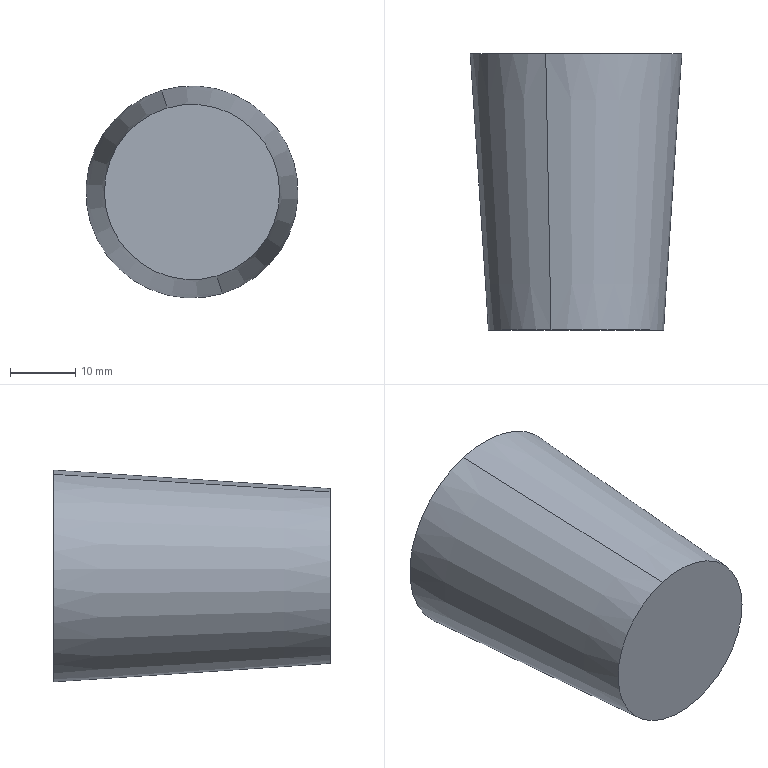Component | SolidWorks | CoffeeCup-1 | 1 solid | 7 faces | box 32.54 x 42.38 x 32.54 mm | volume 8227 mm3 | cone 4 | plane 3
build123d program:
from build123d import *

# Parameters (mm, degrees)
SHELL1_T = -2


with BuildPart() as part:
    # Sketch1 → Revolve1 (revolve)
    with BuildSketch(Plane.XY, mode=Mode.PRIVATE) as revolve1_sk:
        Polygon((0, 0), (16.271, 0), (13.443, -42.384), (0, -42.384), align=None)
    revolve(revolve1_sk.sketch.rotate(Axis((0, -42.384, 0), (0, 1, 0)), 90), axis=Axis((0, -42.384, 0), (0, 1, 0)))

    # Shell1
    shell1_openings = [part.faces().sort_by_distance(p)[0] for p in [
        (0, 0, 0),
    ]]
    offset(amount=SHELL1_T, openings=shell1_openings, kind=Kind.INTERSECTION)


solid = part.part

# Placed as in the assembly
solid = solid.moved(Location((-79.558, -23.012, 243.54), (0, 0, 0)))
STEP:
#1=CARTESIAN_POINT('',(-3.262,-2.496,10.025));
#2=VERTEX_POINT('',#1);
#3=CARTESIAN_POINT('',(-3.002,-2.496,9.152));
#4=VERTEX_POINT('',#3);
#5=CARTESIAN_POINT('',(-3.132,-2.496,9.588));
#6=DIRECTION('',(0.,-1.,0.));
#7=DIRECTION('',(0.2855,0.,-0.9584));
#8=AXIS2_PLACEMENT_3D('',#5,#6,#7);
#9=CIRCLE('',#8,0.4556);
#10=EDGE_CURVE('',#2,#4,#9,.T.);
#11=ORIENTED_EDGE('',*,*,#10,.T.);
#12=CARTESIAN_POINT('',(-2.972,-0.906,9.05));
#13=VERTEX_POINT('',#12);
#14=CARTESIAN_POINT('',(-3.004,-2.569,9.156));
#15=DIRECTION('',(0.01901,0.9978,-0.06379));
#16=VECTOR('',#15,39.37);
#17=LINE('',#14,#16);
#18=EDGE_CURVE('',#4,#13,#17,.T.);
#19=ORIENTED_EDGE('',*,*,#18,.T.);
#20=CARTESIAN_POINT('',(-3.293,-0.906,10.126));
#21=VERTEX_POINT('',#20);
#22=CARTESIAN_POINT('',(-3.132,-0.906,9.588));
#23=DIRECTION('',(0.,-1.,0.));
#24=DIRECTION('',(-0.2855,0.,0.9584));
#25=AXIS2_PLACEMENT_3D('',#22,#23,#24);
#26=CIRCLE('',#25,0.5617);
#27=EDGE_CURVE('',#21,#13,#26,.T.);
#28=ORIENTED_EDGE('',*,*,#27,.F.);
#29=CARTESIAN_POINT('',(-3.261,-2.569,10.02));
#30=DIRECTION('',(-0.01901,0.9978,0.06379));
#31=VECTOR('',#30,39.37);
#32=LINE('',#29,#31);
#33=EDGE_CURVE('',#2,#21,#32,.T.);
#34=ORIENTED_EDGE('',*,*,#33,.F.);
#35=EDGE_LOOP('',(#11,#19,#28,#34));
#36=FACE_OUTER_BOUND('',#35,.T.);
#37=CARTESIAN_POINT('',(-3.132,-2.569,9.588));
#38=DIRECTION('',(0.,1.,0.));
#39=DIRECTION('',(-0.2855,0.,0.9584));
#40=AXIS2_PLACEMENT_3D('',#37,#38,#39);
#41=CONICAL_SURFACE('',#40,0.4507,0.06661);
#42=ADVANCED_FACE('',(#36),#41,.F.);
#43=CARTESIAN_POINT('',(-2.981,-2.575,9.081));
#44=VERTEX_POINT('',#43);
#45=CARTESIAN_POINT('',(-3.283,-2.575,10.095));
#46=VERTEX_POINT('',#45);
#47=CARTESIAN_POINT('',(-3.132,-2.575,9.588));
#48=DIRECTION('',(0.,-1.,0.));
#49=DIRECTION('',(0.2855,0.,-0.9584));
#50=AXIS2_PLACEMENT_3D('',#47,#48,#49);
#51=CIRCLE('',#50,0.5293);
#52=EDGE_CURVE('',#44,#46,#51,.T.);
#53=ORIENTED_EDGE('',*,*,#52,.F.);
#54=CARTESIAN_POINT('',(-2.949,-0.906,8.974));
#55=VERTEX_POINT('',#54);
#56=CARTESIAN_POINT('',(-2.981,-2.575,9.081));
#57=DIRECTION('',(0.01901,0.9978,-0.06379));
#58=VECTOR('',#57,39.37);
#59=LINE('',#56,#58);
#60=EDGE_CURVE('',#44,#55,#59,.T.);
#61=ORIENTED_EDGE('',*,*,#60,.T.);
#62=CARTESIAN_POINT('',(-3.315,-0.906,10.202));
#63=VERTEX_POINT('',#62);
#64=CARTESIAN_POINT('',(-3.132,-0.906,9.588));
#65=DIRECTION('',(0.,-1.,0.));
#66=DIRECTION('',(0.2855,0.,-0.9584));
#67=AXIS2_PLACEMENT_3D('',#64,#65,#66);
#68=CIRCLE('',#67,0.6406);
#69=EDGE_CURVE('',#55,#63,#68,.T.);
#70=ORIENTED_EDGE('',*,*,#69,.T.);
#71=CARTESIAN_POINT('',(-3.283,-2.575,10.095));
#72=DIRECTION('',(-0.01901,0.9978,0.06379));
#73=VECTOR('',#72,39.37);
#74=LINE('',#71,#73);
#75=EDGE_CURVE('',#46,#63,#74,.T.);
#76=ORIENTED_EDGE('',*,*,#75,.F.);
#77=EDGE_LOOP('',(#53,#61,#70,#76));
#78=FACE_OUTER_BOUND('',#77,.T.);
#79=CARTESIAN_POINT('',(-3.132,-2.575,9.588));
#80=DIRECTION('',(0.,1.,0.));
#81=DIRECTION('',(-0.2855,0.,0.9584));
#82=AXIS2_PLACEMENT_3D('',#79,#80,#81);
#83=CONICAL_SURFACE('',#82,0.5293,0.06661);
#84=ADVANCED_FACE('',(#78),#83,.T.);
#85=ORIENTED_EDGE('',*,*,#27,.T.);
#86=CARTESIAN_POINT('',(-3.132,-0.906,9.588));
#87=DIRECTION('',(0.,-1.,0.));
#88=DIRECTION('',(-0.2855,0.,0.9584));
#89=AXIS2_PLACEMENT_3D('',#86,#87,#88);
#90=CIRCLE('',#89,0.5617);
#91=EDGE_CURVE('',#13,#21,#90,.T.);
#92=ORIENTED_EDGE('',*,*,#91,.T.);
#93=EDGE_LOOP('',(#85,#92));
#94=FACE_BOUND('',#93,.T.);
#95=CARTESIAN_POINT('',(-3.132,-0.906,9.588));
#96=DIRECTION('',(0.,-1.,0.));
#97=DIRECTION('',(0.2855,0.,-0.9584));
#98=AXIS2_PLACEMENT_3D('',#95,#96,#97);
#99=CIRCLE('',#98,0.6406);
#100=EDGE_CURVE('',#63,#55,#99,.T.);
#101=ORIENTED_EDGE('',*,*,#100,.F.);
#102=ORIENTED_EDGE('',*,*,#69,.F.);
#103=EDGE_LOOP('',(#101,#102));
#104=FACE_OUTER_BOUND('',#103,.T.);
#105=CARTESIAN_POINT('',(-3.132,-0.906,9.588));
#106=DIRECTION('',(0.,1.,0.));
#107=DIRECTION('',(-0.2855,0.,0.9584));
#108=AXIS2_PLACEMENT_3D('',#105,#106,#107);
#109=PLANE('',#108);
#110=ADVANCED_FACE('',(#94,#104),#109,.T.);
#111=ORIENTED_EDGE('',*,*,#60,.F.);
#112=CARTESIAN_POINT('',(-3.132,-2.575,9.588));
#113=DIRECTION('',(0.,-1.,0.));
#114=DIRECTION('',(0.2855,0.,-0.9584));
#115=AXIS2_PLACEMENT_3D('',#112,#113,#114);
#116=CIRCLE('',#115,0.5293);
#117=EDGE_CURVE('',#46,#44,#116,.T.);
#118=ORIENTED_EDGE('',*,*,#117,.F.);
#119=ORIENTED_EDGE('',*,*,#75,.T.);
#120=ORIENTED_EDGE('',*,*,#100,.T.);
#121=EDGE_LOOP('',(#111,#118,#119,#120));
#122=FACE_OUTER_BOUND('',#121,.T.);
#123=CARTESIAN_POINT('',(-3.132,-2.575,9.588));
#124=DIRECTION('',(0.,1.,0.));
#125=DIRECTION('',(-0.2855,0.,0.9584));
#126=AXIS2_PLACEMENT_3D('',#123,#124,#125);
#127=CONICAL_SURFACE('',#126,0.5293,0.06661);
#128=ADVANCED_FACE('',(#122),#127,.T.);
#129=ORIENTED_EDGE('',*,*,#117,.T.);
#130=ORIENTED_EDGE('',*,*,#52,.T.);
#131=EDGE_LOOP('',(#129,#130));
#132=FACE_OUTER_BOUND('',#131,.T.);
#133=CARTESIAN_POINT('',(-2.625,-2.575,9.739));
#134=DIRECTION('',(0.,-1.,0.));
#135=DIRECTION('',(0.2855,0.,-0.9584));
#136=AXIS2_PLACEMENT_3D('',#133,#134,#135);
#137=PLANE('',#136);
#138=ADVANCED_FACE('',(#132),#137,.T.);
#139=ORIENTED_EDGE('',*,*,#18,.F.);
#140=CARTESIAN_POINT('',(-3.132,-2.496,9.588));
#141=DIRECTION('',(0.,-1.,0.));
#142=DIRECTION('',(0.2855,0.,-0.9584));
#143=AXIS2_PLACEMENT_3D('',#140,#141,#142);
#144=CIRCLE('',#143,0.4556);
#145=EDGE_CURVE('',#4,#2,#144,.T.);
#146=ORIENTED_EDGE('',*,*,#145,.T.);
#147=ORIENTED_EDGE('',*,*,#33,.T.);
#148=ORIENTED_EDGE('',*,*,#91,.F.);
#149=EDGE_LOOP('',(#139,#146,#147,#148));
#150=FACE_OUTER_BOUND('',#149,.T.);
#151=CARTESIAN_POINT('',(-3.132,-2.569,9.588));
#152=DIRECTION('',(0.,1.,0.));
#153=DIRECTION('',(-0.2855,0.,0.9584));
#154=AXIS2_PLACEMENT_3D('',#151,#152,#153);
#155=CONICAL_SURFACE('',#154,0.4507,0.06661);
#156=ADVANCED_FACE('',(#150),#155,.F.);
#157=ORIENTED_EDGE('',*,*,#10,.F.);
#158=ORIENTED_EDGE('',*,*,#145,.F.);
#159=EDGE_LOOP('',(#157,#158));
#160=FACE_OUTER_BOUND('',#159,.T.);
#161=CARTESIAN_POINT('',(-2.625,-2.496,9.739));
#162=DIRECTION('',(0.,-1.,0.));
#163=DIRECTION('',(0.2855,0.,-0.9584));
#164=AXIS2_PLACEMENT_3D('',#161,#162,#163);
#165=PLANE('',#164);
#166=ADVANCED_FACE('',(#160),#165,.F.);
#167=CLOSED_SHELL('',(#42,#84,#110,#128,#138,#156,#166));
#168=MANIFOLD_SOLID_BREP('',#167);
#169=CARTESIAN_POINT('',(0.,0.,0.));
#170=DIRECTION('',(0.,0.,1.));
#171=DIRECTION('',(1.,0.,0.));
#172=AXIS2_PLACEMENT_3D('',#169,#170,#171);
#173=(LENGTH_UNIT()NAMED_UNIT(*)SI_UNIT($,.METRE.));
#174=LENGTH_MEASURE_WITH_UNIT(LENGTH_MEASURE(0.0254),#173);
#175=DIMENSIONAL_EXPONENTS(1.,0.,0.,0.,0.,0.,0.);
#176=(CONVERSION_BASED_UNIT('',#174)LENGTH_UNIT()NAMED_UNIT(#175));
#177=UNCERTAINTY_MEASURE_WITH_UNIT(LENGTH_MEASURE(0.00001),#176,'','');
#178=(NAMED_UNIT(*)PLANE_ANGLE_UNIT()SI_UNIT($,.RADIAN.));
#179=(NAMED_UNIT(*)SI_UNIT($,.STERADIAN.)SOLID_ANGLE_UNIT());
#180=(GEOMETRIC_REPRESENTATION_CONTEXT(3)GLOBAL_UNCERTAINTY_ASSIGNED_CONTEXT((#177))GLOBAL_UNIT_ASSIGNED_CONTEXT((#176,#178,#179))REPRESENTATION_CONTEXT('',''));
#181=ADVANCED_BREP_SHAPE_REPRESENTATION('',(#168,#172),#180);
#182=COLOUR_RGB('',0.7922,0.8196,0.9333);
#183=FILL_AREA_STYLE_COLOUR('',#182);
#184=FILL_AREA_STYLE('',(#183));
#185=SURFACE_STYLE_FILL_AREA(#184);
#186=SURFACE_SIDE_STYLE('',(#185));
#187=SURFACE_STYLE_USAGE(.BOTH.,#186);
#188=PRESENTATION_STYLE_ASSIGNMENT((#187));
#189=STYLED_ITEM('',(#188),#168);
#190=PRESENTATION_LAYER_ASSIGNMENT('','',(#189));
#191=(LENGTH_UNIT()NAMED_UNIT(*)SI_UNIT($,.METRE.));
#192=LENGTH_MEASURE_WITH_UNIT(LENGTH_MEASURE(0.0254),#191);
#193=DIMENSIONAL_EXPONENTS(1.,0.,0.,0.,0.,0.,0.);
#194=(CONVERSION_BASED_UNIT('',#192)LENGTH_UNIT()NAMED_UNIT(#193));
#195=UNCERTAINTY_MEASURE_WITH_UNIT(LENGTH_MEASURE(0.00001),#194,'','');
#196=(NAMED_UNIT(*)PLANE_ANGLE_UNIT()SI_UNIT($,.RADIAN.));
#197=(NAMED_UNIT(*)SI_UNIT($,.STERADIAN.)SOLID_ANGLE_UNIT());
#198=(GEOMETRIC_REPRESENTATION_CONTEXT(3)GLOBAL_UNCERTAINTY_ASSIGNED_CONTEXT((#195))GLOBAL_UNIT_ASSIGNED_CONTEXT((#194,#196,#197))REPRESENTATION_CONTEXT('',''));
#199=MECHANICAL_DESIGN_GEOMETRIC_PRESENTATION_REPRESENTATION('',(#189),#198);